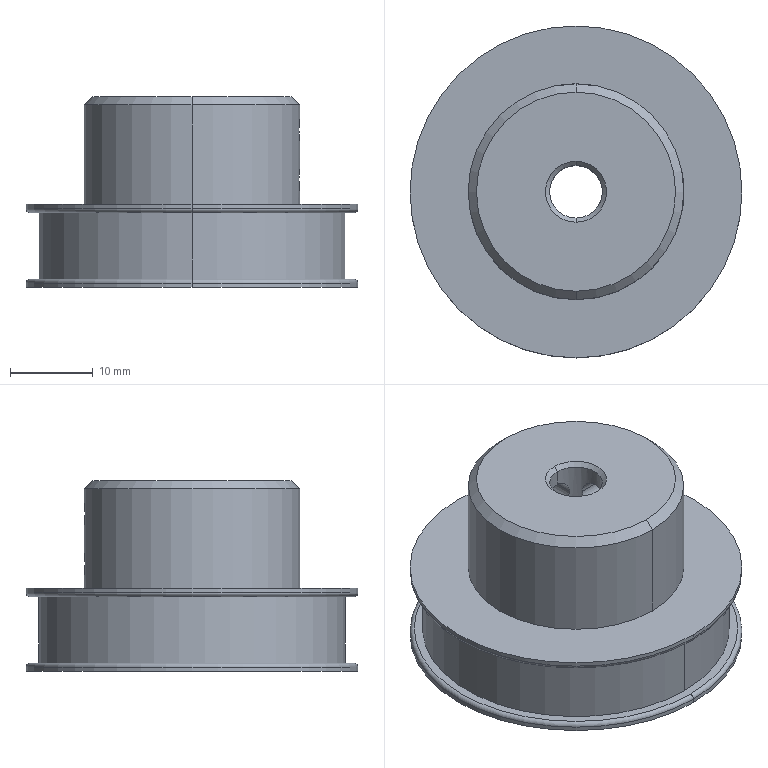Component | SolidWorks | SL010-RightStreamline-1-1_SL010-BeltMotorAssembly-1-1_SL010-0ALk-010000-006-2-1-1 | 1 solid | 33 faces | box 40 x 40 x 23 mm | volume 16891 mm3 | cylinder 18 | cone 6 | plane 5 | torus 4 | commonest cylinder face diameters 3.3 x8 40 x4 37 x2 6.35 x2 26 x2 | material 45
build123d program:
from build123d import *

# Parameters (mm, degrees)
SKETCH1_R                  = 13
BOSS_EXTRUDE1_DEPTH        = 13
SKETCH2_R                  = 20
BOSS_EXTRUDE2_DEPTH        = 10
SKETCH3_R                  = 3.175
CUT_EXTRUDE1_DEPTH         = 37.455
SKETCH4_W                  = 1.5
SKETCH4_H                  = 8
FILLET1_R                  = 0.5
M4_TAPPED_HOLE1_AT_2_COUNT = 2
M4_TAPPED_HOLE1_AT_2_PITCH = 6
CHAMFER1_SIZE              = 1
CHAMFER2_SIZE              = 0.5
CIRPATTERN1_COUNT          = 2
CIRPATTERN1_ANGLE          = 90


with BuildPart() as part:
    # Sketch1 → Boss-Extrude1 (new body)
    with BuildSketch(Plane(origin=(0, 0, 0), x_dir=(1, 0, 0), z_dir=(0, 1, 0))):
        with Locations(Location((0, 0, 0), (0, 0, 90))):
            Circle(SKETCH1_R)
    extrude(amount=BOSS_EXTRUDE1_DEPTH)

    # Sketch2 → Boss-Extrude2 (add)
    with BuildSketch(Plane.XZ):
        with Locations(Location((0, 0, 0), (0, 0, 270))):
            Circle(SKETCH2_R)
    extrude(amount=BOSS_EXTRUDE2_DEPTH)

    # Sketch3 → Cut-Extrude1 (cut, through all)
    with BuildSketch(Plane(origin=(0, 13, 0), x_dir=(1, 0, 0), z_dir=(0, 1, 0))):
        with Locations(Location((0, 0, 0), (0, 0, 270))):
            Circle(SKETCH3_R)
    extrude(amount=-CUT_EXTRUDE1_DEPTH, mode=Mode.SUBTRACT)

    # Sketch4 → Cut-Revolve1 (revolve, cut)
    with BuildSketch(Plane.XY, mode=Mode.PRIVATE) as cut_revolve1_sk:
        with Locations((-19.25, -5)):
            Rectangle(SKETCH4_W, SKETCH4_H)
    revolve(cut_revolve1_sk.sketch.rotate(Axis((0, 0, 0), (0, -1, 0)), 270), axis=Axis((0, 0, 0), (0, -1, 0)), mode=Mode.SUBTRACT)

    # Fillet1
    fillet1_edges = [part.edges().sort_by_distance(p)[0] for p in [
        (0, -9, 20),
        (0, -1, 20),
    ]]
    fillet(fillet1_edges, radius=FILLET1_R)

    # Sketch5 → M4 Tapped Hole1 (revolve, cut)
    with BuildSketch(Plane(origin=(0, 9, 13), x_dir=(0, -1, 0), z_dir=(1, 0, 0))):
        Polygon((0, 0), (0, 11.491), (1.65, 10.5), (1.65, 0), align=None)
    m4_tapped_hole1 = revolve(axis=Axis((0, 9, 19.35), (0, 0, -1)), mode=Mode.SUBTRACT)

    # M4 Tapped Hole1 at 2: M4 Tapped Hole1 ×2
    with Locations(*[(0, -i * M4_TAPPED_HOLE1_AT_2_PITCH, 0) for i in range(1, M4_TAPPED_HOLE1_AT_2_COUNT)]):
        add(m4_tapped_hole1, mode=Mode.SUBTRACT)

    # Chamfer1
    chamfer1_edges = [part.edges().sort_by_distance(p)[0] for p in [
        (0, 13, 13),
    ]]
    chamfer(chamfer1_edges, length=CHAMFER1_SIZE)

    # Chamfer2
    chamfer2_edges = [part.edges().sort_by_distance(p)[0] for p in [
        (0, -10, -3.175),
        (0, 13, -3.175),
    ]]
    chamfer(chamfer2_edges, length=CHAMFER2_SIZE)

    # CirPattern1: M4 Tapped Hole1 ×2 about axis
    cirpattern1_axis = Axis((0, 13, 0), (0, -1, 0))
    for i in range(1, CIRPATTERN1_COUNT):
        add(m4_tapped_hole1.rotate(cirpattern1_axis, i * CIRPATTERN1_ANGLE / (CIRPATTERN1_COUNT - 1)), mode=Mode.SUBTRACT)

    # CirPattern1 copy 1 sketch → CirPattern1 copy 1 (revolve, cut)
    with BuildSketch(Plane(origin=(-13, 3, 0), x_dir=(0, -1, 0), z_dir=(0, 0, 1))):
        Polygon((0, 0), (0, 11.491), (1.65, 10.5), (1.65, 0), align=None)
    revolve(axis=Axis((-19.35, 3, 0), (1, 0, 0)), mode=Mode.SUBTRACT)


solid = part.part

# Placed as in the assembly
solid = solid.moved(Location((-580, -191.454, -305.235), (-90, 0, 180)))